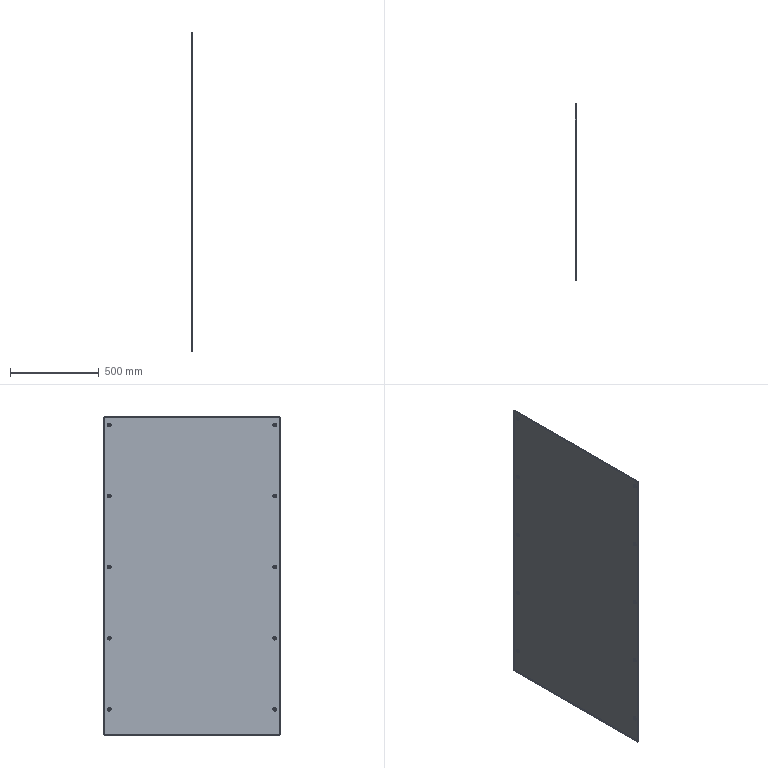Component | SolidWorks | HighVoltageOuterSealingPlate-1 | 1 solid | 118 faces | volume 2169335 mm3 | plane 42 | cone 40 | cylinder 28 | spline 8 | commonest cylinder face diameters 7 x20 1.473 x4 3.873 x4 | material Plain Carbon Steel